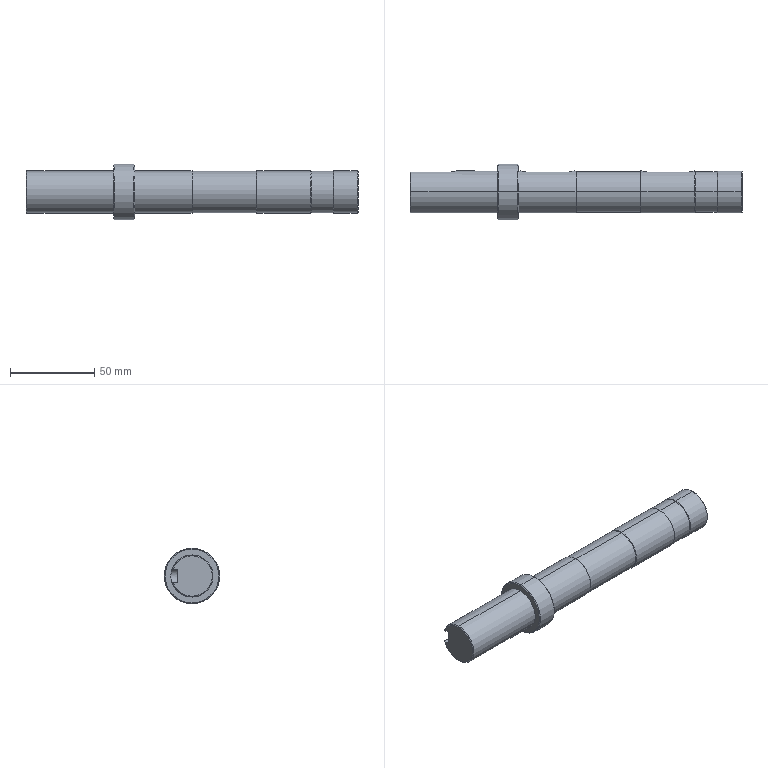CAM job | Mastercam | mm | 2 operations | part box 197 x 33 x 33
1. Contour (Ramp) | 5 - 6 平铣刀
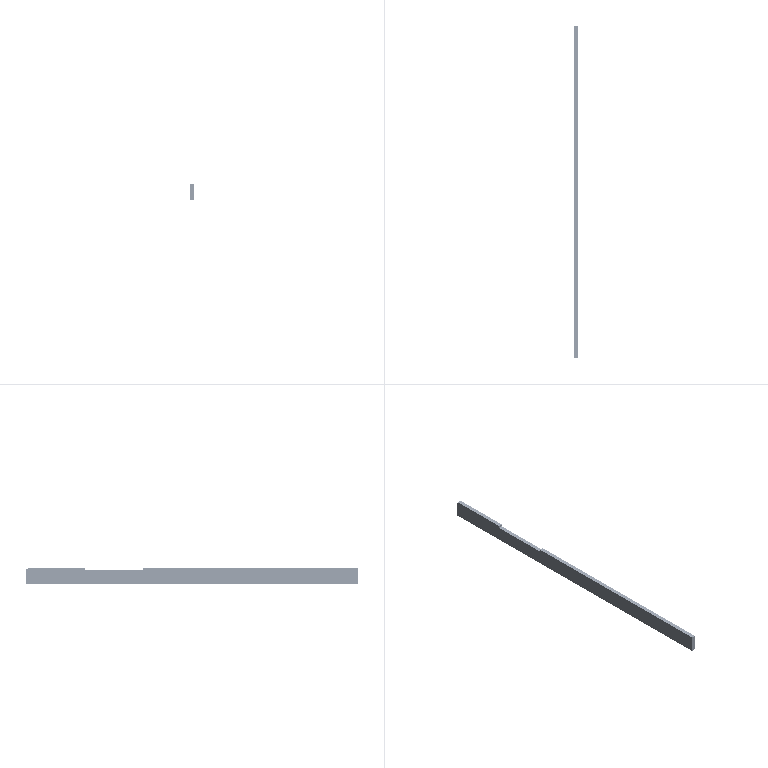2. Contour (Ramp) | 5 - 6 平铣刀